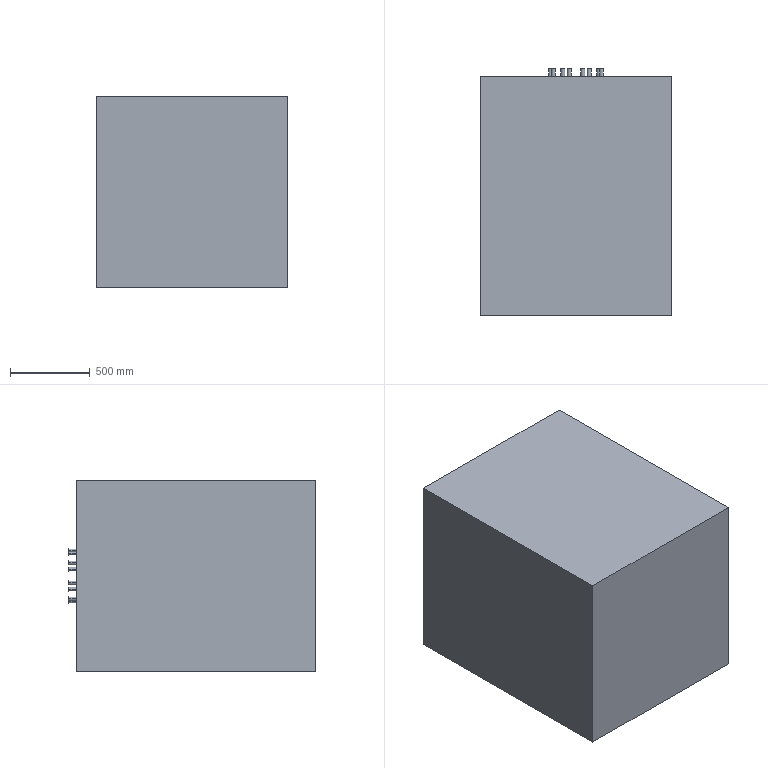Component | SolidWorks | Base-1 | 1 solid | 46 faces | box 1200 x 1550 x 1200 mm | volume 2160179816 mm3 | cone 16 | cylinder 16 | plane 14 | commonest cylinder face diameters 24 x16
build123d program:
from build123d import *

# Parameters (mm, degrees)
SKETCH1_W           = 1200
SKETCH1_H           = 1200
BOSS_EXTRUDE1_DEPTH = 1500
SKETCH2_R           = 12
BOSS_EXTRUDE2_DEPTH = 50
CIRPATTERN1_COUNT   = 8
CHAMFER1_SIZE       = 2


with BuildPart() as part:
    # Sketch1 → Boss-Extrude1 (new body)
    with BuildSketch(Plane.XY):
        Rectangle(SKETCH1_W, SKETCH1_H)
    extrude(amount=BOSS_EXTRUDE1_DEPTH)

    # Sketch2 → Boss-Extrude2 (add)
    with BuildSketch(Plane(origin=(0, 0, 0), x_dir=(-1, 0, 0), z_dir=(0, 0, -1))):
        with Locations(Location((-142.894, -82.5, 0), (0, 0, 180))):
            Circle(SKETCH2_R)
    boss_extrude2 = extrude(amount=BOSS_EXTRUDE2_DEPTH)

    # CirPattern1: Boss-Extrude2 ×8 about axis
    cirpattern1_axis = Axis((0, 0, 0), (0, 0, 1))
    for i in range(1, CIRPATTERN1_COUNT):
        add(boss_extrude2.rotate(cirpattern1_axis, i * 360 / CIRPATTERN1_COUNT))

    # Chamfer1
    chamfer1_edges = [part.edges().sort_by_distance(p)[0] for p in [
        (130.894, -82.5, -50),
        (34.22, -150.892, -50),
        (-82.5, -130.894, -50),
        (-150.892, -34.22, -50),
        (-130.894, 82.5, -50),
        (-34.22, 150.892, -50),
        (82.5, 130.894, -50),
        (150.892, 34.22, -50),
    ]]
    chamfer(chamfer1_edges, length=CHAMFER1_SIZE)


solid = part.part

# Placed as in the assembly
solid = solid.moved(Location((0, 0, 0), (90, 0, 0)))